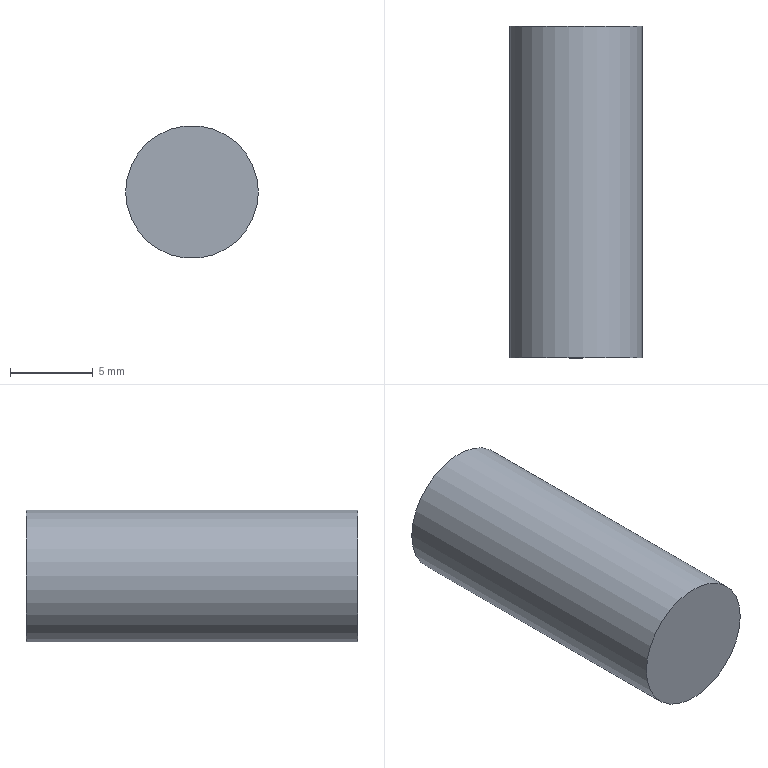Component | NX | FRONT_WHEEL_AXLE | 1 solid | 3 faces | box 8 x 20 x 8 mm | volume 1005 mm3 | plane 2 | cylinder 1 | commonest cylinder face diameters 8 x1
STEP:
#1=CARTESIAN_POINT('',(0.,0.,0.));
#2=DIRECTION('',(0.,0.,1.));
#3=DIRECTION('',(1.,0.,0.));
#4=AXIS2_PLACEMENT_3D('',#1,#2,#3);
#5=CARTESIAN_POINT('',(-189.955,10.,-58.));
#6=VERTEX_POINT('',#5);
#7=CARTESIAN_POINT('',(-193.955,10.,-58.));
#8=DIRECTION('',(0.,-1.,0.));
#9=DIRECTION('',(1.,0.,0.));
#10=AXIS2_PLACEMENT_3D('',#7,#8,#9);
#11=CIRCLE('',#10,4.);
#12=CARTESIAN_POINT('',(-193.955,10.,-58.));
#13=DIRECTION('',(0.,-1.,0.));
#14=DIRECTION('',(-1.,0.,0.));
#15=AXIS2_PLACEMENT_3D('',#12,#13,#14);
#16=CYLINDRICAL_SURFACE('',#15,4.);
#17=CARTESIAN_POINT('',(3.142,0.));
#18=DIRECTION('',(1.,0.));
#19=VECTOR('',#18,1.);
#20=LINE('',#17,#19);
#21=(GEOMETRIC_REPRESENTATION_CONTEXT(2)PARAMETRIC_REPRESENTATION_CONTEXT()REPRESENTATION_CONTEXT('',''));
#22=DEFINITIONAL_REPRESENTATION('',(#20),#21);
#23=PCURVE('',#16,#22);
#24=CARTESIAN_POINT('',(-193.955,10.,-58.));
#25=DIRECTION('',(0.,-1.,0.));
#26=DIRECTION('',(-1.,0.,0.));
#27=AXIS2_PLACEMENT_3D('',#24,#25,#26);
#28=PLANE('',#27);
#29=CARTESIAN_POINT('',(0.,0.));
#30=DIRECTION('',(-1.,0.));
#31=AXIS2_PLACEMENT_2D('',#29,#30);
#32=CIRCLE('',#31,4.);
#33=(GEOMETRIC_REPRESENTATION_CONTEXT(2)PARAMETRIC_REPRESENTATION_CONTEXT()REPRESENTATION_CONTEXT('',''));
#34=DEFINITIONAL_REPRESENTATION('',(#32),#33);
#35=PCURVE('',#28,#34);
#36=SURFACE_CURVE('',#11,(#23,#35),.PCURVE_S1.);
#37=EDGE_CURVE('',#6,#6,#36,.T.);
#38=ORIENTED_EDGE('',*,*,#37,.T.);
#39=CARTESIAN_POINT('',(-189.955,-10.,-58.));
#40=VERTEX_POINT('',#39);
#41=CARTESIAN_POINT('',(-189.955,10.,-58.));
#42=CARTESIAN_POINT('',(-189.955,-10.,-58.));
#43=B_SPLINE_CURVE_WITH_KNOTS('',1,(#41,#42),.UNSPECIFIED.,.F.,.F.,(2,2),(0.,20.),.PIECEWISE_BEZIER_KNOTS.);
#44=CARTESIAN_POINT('',(9.425,0.));
#45=DIRECTION('',(0.,1.));
#46=VECTOR('',#45,1.);
#47=LINE('',#44,#46);
#48=(GEOMETRIC_REPRESENTATION_CONTEXT(2)PARAMETRIC_REPRESENTATION_CONTEXT()REPRESENTATION_CONTEXT('',''));
#49=DEFINITIONAL_REPRESENTATION('',(#47),#48);
#50=PCURVE('',#16,#49);
#51=CARTESIAN_POINT('',(3.142,0.));
#52=DIRECTION('',(0.,1.));
#53=VECTOR('',#52,1.);
#54=LINE('',#51,#53);
#55=(GEOMETRIC_REPRESENTATION_CONTEXT(2)PARAMETRIC_REPRESENTATION_CONTEXT()REPRESENTATION_CONTEXT('',''));
#56=DEFINITIONAL_REPRESENTATION('',(#54),#55);
#57=PCURVE('',#16,#56);
#58=SEAM_CURVE('',#43,(#50,#57),.PCURVE_S1.);
#59=EDGE_CURVE('',#6,#40,#58,.T.);
#60=ORIENTED_EDGE('',*,*,#59,.T.);
#61=CARTESIAN_POINT('',(-193.955,-10.,-58.));
#62=DIRECTION('',(0.,-1.,0.));
#63=DIRECTION('',(1.,0.,0.));
#64=AXIS2_PLACEMENT_3D('',#61,#62,#63);
#65=CIRCLE('',#64,4.);
#66=CARTESIAN_POINT('',(3.142,20.));
#67=DIRECTION('',(1.,0.));
#68=VECTOR('',#67,1.);
#69=LINE('',#66,#68);
#70=(GEOMETRIC_REPRESENTATION_CONTEXT(2)PARAMETRIC_REPRESENTATION_CONTEXT()REPRESENTATION_CONTEXT('',''));
#71=DEFINITIONAL_REPRESENTATION('',(#69),#70);
#72=PCURVE('',#16,#71);
#73=CARTESIAN_POINT('',(-193.955,-10.,-58.));
#74=DIRECTION('',(0.,-1.,0.));
#75=DIRECTION('',(-1.,0.,0.));
#76=AXIS2_PLACEMENT_3D('',#73,#74,#75);
#77=PLANE('',#76);
#78=CARTESIAN_POINT('',(0.,0.));
#79=DIRECTION('',(-1.,0.));
#80=AXIS2_PLACEMENT_2D('',#78,#79);
#81=CIRCLE('',#80,4.);
#82=(GEOMETRIC_REPRESENTATION_CONTEXT(2)PARAMETRIC_REPRESENTATION_CONTEXT()REPRESENTATION_CONTEXT('',''));
#83=DEFINITIONAL_REPRESENTATION('',(#81),#82);
#84=PCURVE('',#77,#83);
#85=SURFACE_CURVE('',#65,(#72,#84),.PCURVE_S1.);
#86=EDGE_CURVE('',#40,#40,#85,.T.);
#87=ORIENTED_EDGE('',*,*,#86,.F.);
#88=ORIENTED_EDGE('',*,*,#59,.F.);
#89=EDGE_LOOP('',(#38,#60,#87,#88));
#90=FACE_BOUND('',#89,.T.);
#91=ADVANCED_FACE('',(#90),#16,.T.);
#92=ORIENTED_EDGE('',*,*,#37,.F.);
#93=EDGE_LOOP('',(#92));
#94=FACE_BOUND('',#93,.T.);
#95=ADVANCED_FACE('',(#94),#28,.F.);
#96=ORIENTED_EDGE('',*,*,#86,.T.);
#97=EDGE_LOOP('',(#96));
#98=FACE_BOUND('',#97,.T.);
#99=ADVANCED_FACE('',(#98),#77,.T.);
#100=CLOSED_SHELL('',(#91,#95,#99));
#101=MANIFOLD_SOLID_BREP('',#100);
#102=(LENGTH_UNIT()NAMED_UNIT(*)SI_UNIT(.MILLI.,.METRE.));
#103=UNCERTAINTY_MEASURE_WITH_UNIT(LENGTH_MEASURE(0.00001),#102,'','');
#104=(NAMED_UNIT(*)PLANE_ANGLE_UNIT()SI_UNIT($,.RADIAN.));
#105=(NAMED_UNIT(*)SI_UNIT($,.STERADIAN.)SOLID_ANGLE_UNIT());
#106=(GEOMETRIC_REPRESENTATION_CONTEXT(3)GLOBAL_UNCERTAINTY_ASSIGNED_CONTEXT((#103))GLOBAL_UNIT_ASSIGNED_CONTEXT((#102,#104,#105))REPRESENTATION_CONTEXT('',''));
#107=ADVANCED_BREP_SHAPE_REPRESENTATION('',(#4,#101),#106);